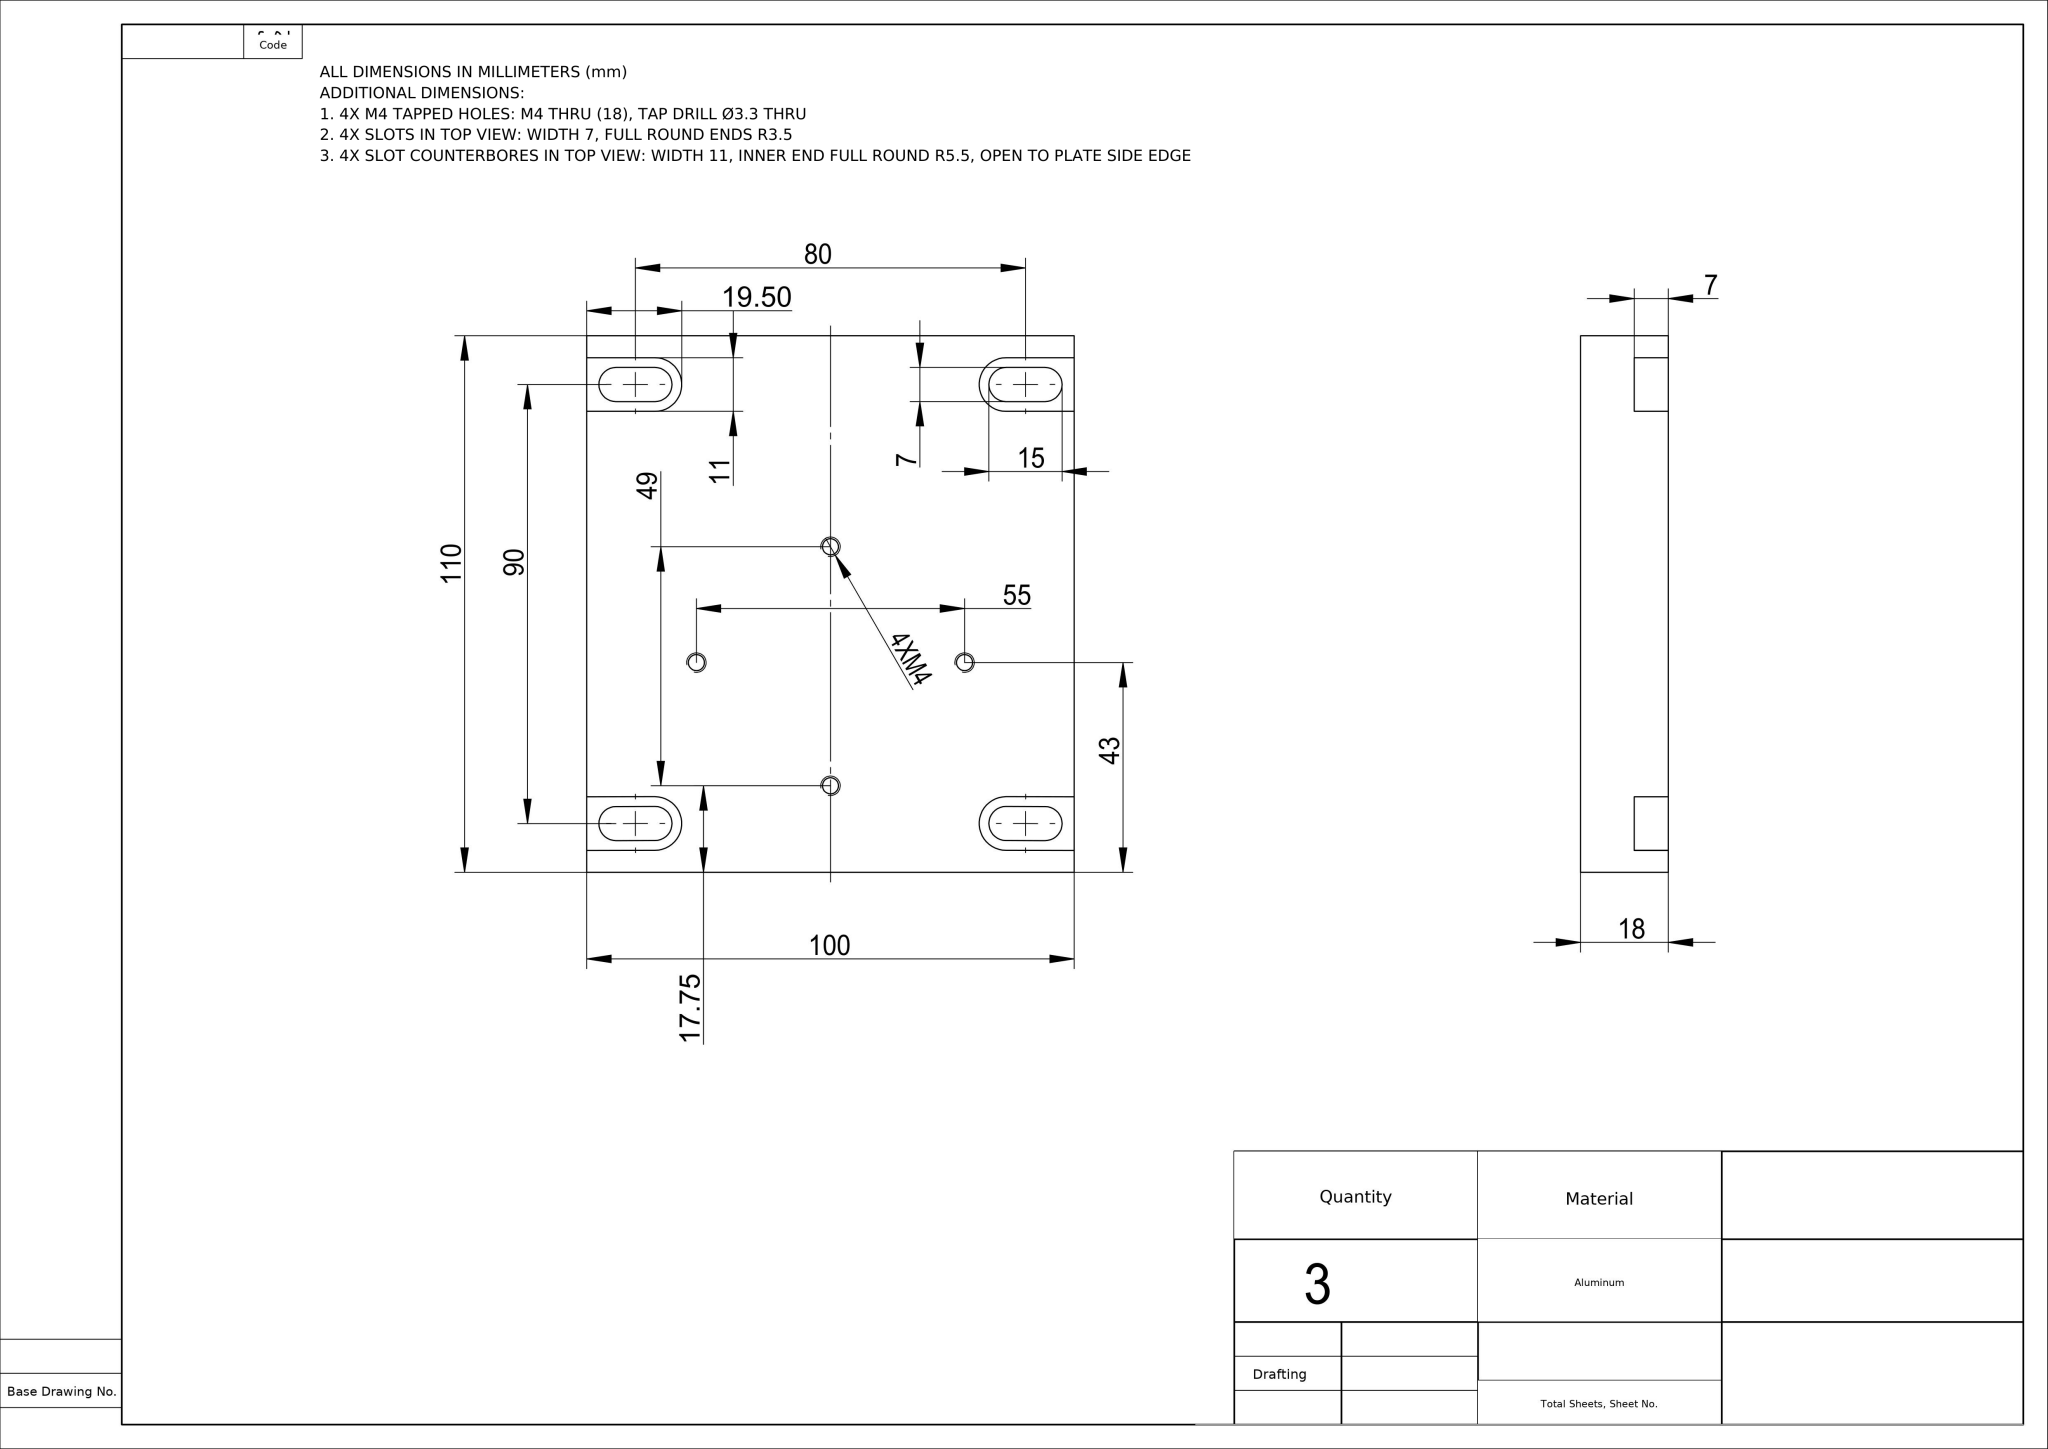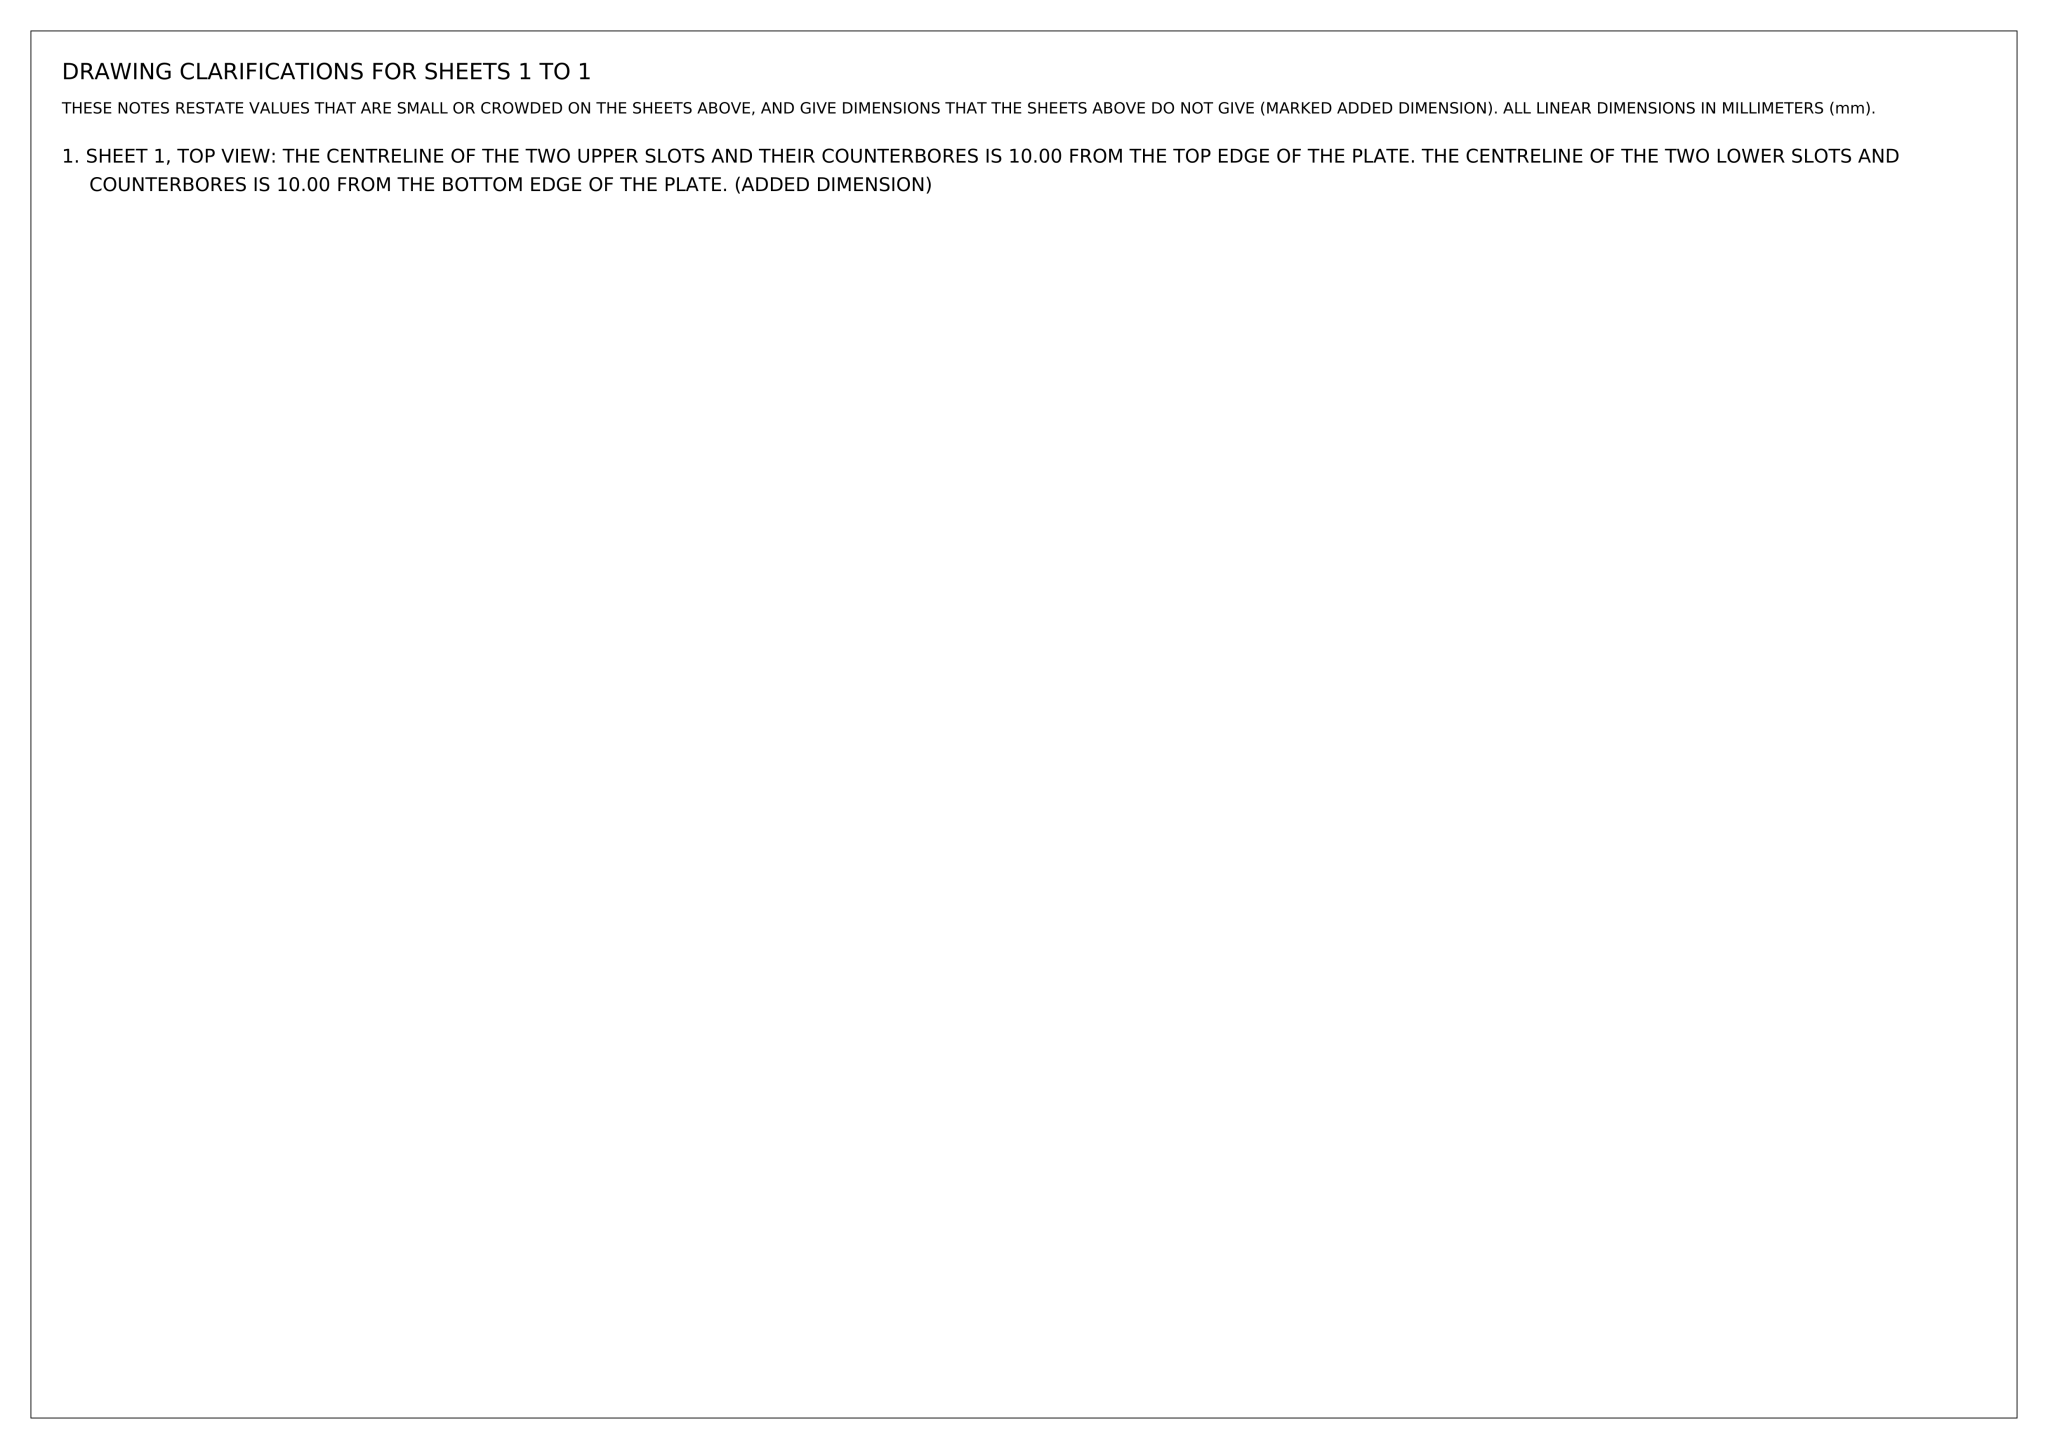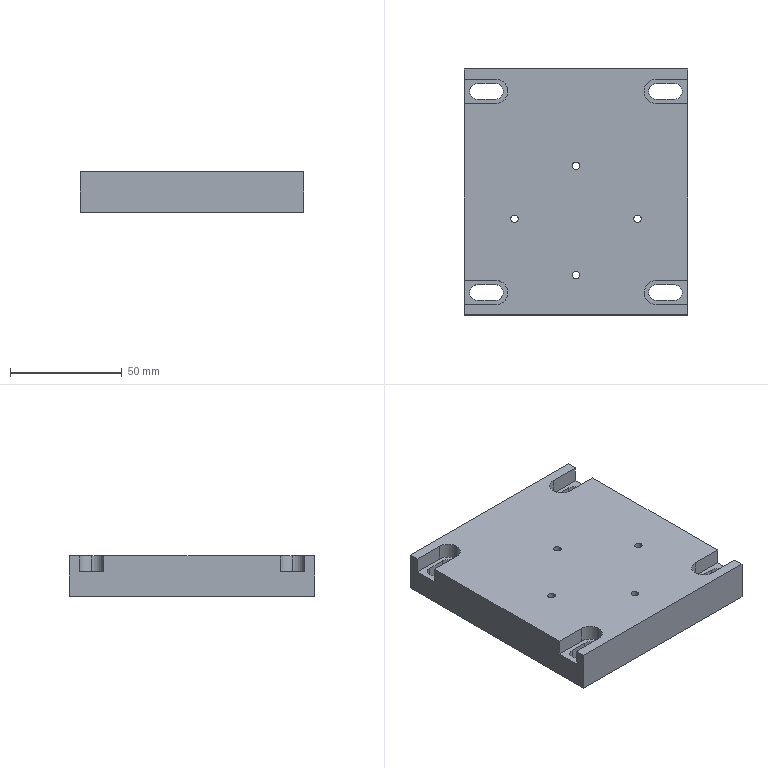Part | NX | mm | 1 solid | 52 faces | box 100 x 110 x 18 mm | volume 187584 mm3 | cylinder 26 | plane 26 | commonest cylinder face diameters 7 x12 3.3 x8 11 x6